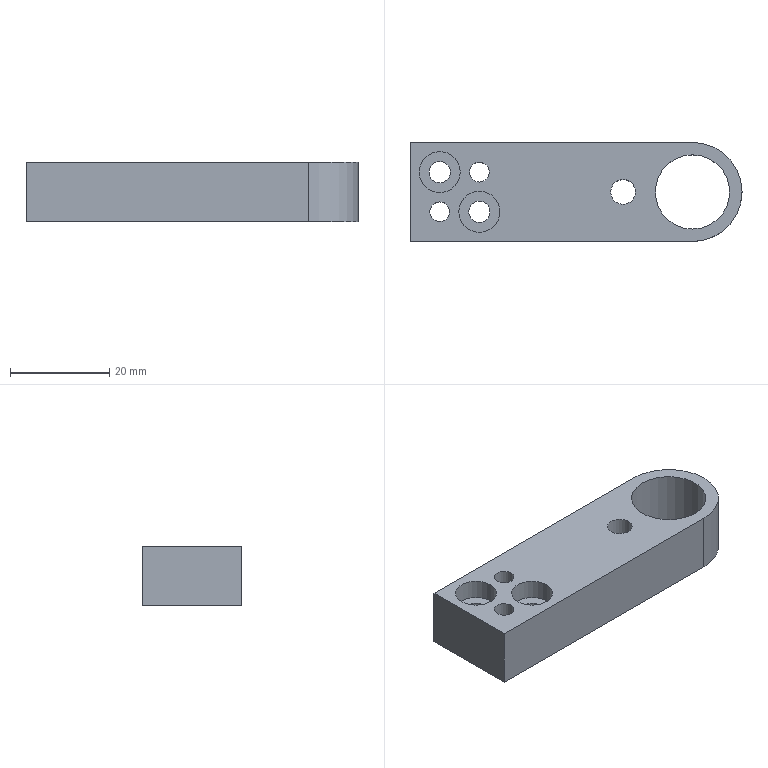Component | NX | DRILL_TEMPLATE | 1 solid | 16 faces | volume 12242 mm3 | cylinder 9 | plane 7 | commonest cylinder face diameters 4.3 x2 4 x2 8.3 x2 20 x1 15 x1 5 x1